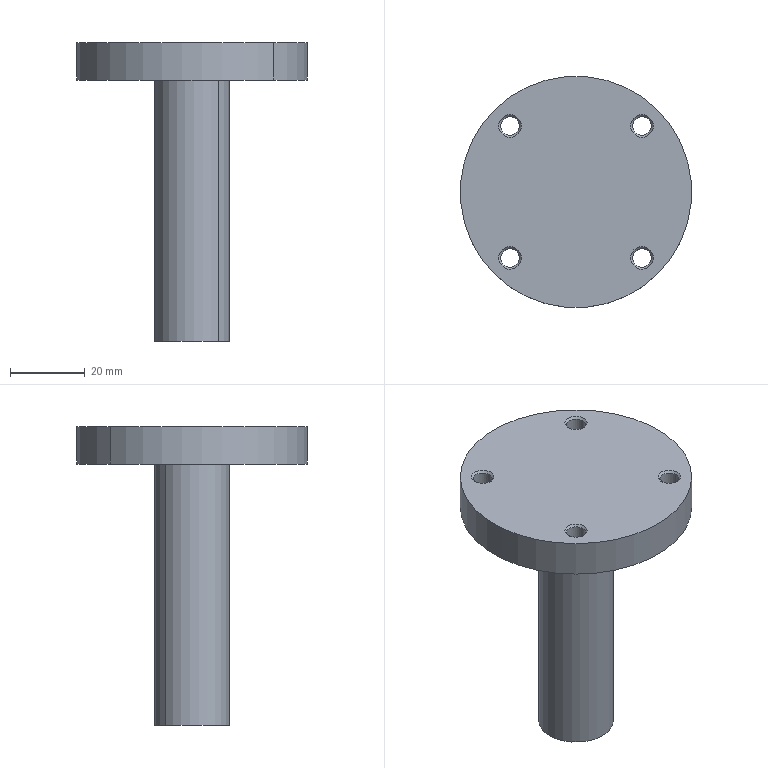Component | SolidWorks | ConnectingBase-3 | 1 solid | 23 faces | box 62 x 62 x 80 mm | volume 51387 mm3 | cylinder 12 | cone 8 | plane 3 | commonest cylinder face diameters 5 x8 20 x2 62 x2
STEP:
#1=COLOUR_RGB('',0.7922,0.8196,0.9333);
#2=FILL_AREA_STYLE_COLOUR('',#1);
#3=FILL_AREA_STYLE('',(#2));
#4=SURFACE_STYLE_FILL_AREA(#3);
#5=SURFACE_SIDE_STYLE('',(#4));
#6=SURFACE_STYLE_USAGE(.BOTH.,#5);
#7=PRESENTATION_STYLE_ASSIGNMENT((#6));
#8=CARTESIAN_POINT('',(-0.4155,17.384,-10.946));
#9=VERTEX_POINT('',#8);
#10=CARTESIAN_POINT('',(-0.5547,17.523,-10.946));
#11=VERTEX_POINT('',#10);
#12=CARTESIAN_POINT('',(-0.4851,17.454,-10.946));
#13=DIRECTION('',(-0.,-0.,1.));
#14=DIRECTION('',(-0.7071,0.7071,0.));
#15=AXIS2_PLACEMENT_3D('',#12,#13,#14);
#16=CIRCLE('',#15,0.09843);
#17=EDGE_CURVE('',#9,#11,#16,.T.);
#18=ORIENTED_EDGE('',*,*,#17,.F.);
#19=CARTESIAN_POINT('',(-0.4009,17.369,-10.925));
#20=VERTEX_POINT('',#19);
#21=CARTESIAN_POINT('',(-0.4155,17.384,-10.946));
#22=DIRECTION('',(0.5,-0.5,0.7071));
#23=VECTOR('',#22,39.37);
#24=LINE('',#21,#23);
#25=EDGE_CURVE('',#9,#20,#24,.T.);
#26=ORIENTED_EDGE('',*,*,#25,.T.);
#27=CARTESIAN_POINT('',(-0.5693,17.538,-10.925));
#28=VERTEX_POINT('',#27);
#29=CARTESIAN_POINT('',(-0.4851,17.454,-10.925));
#30=DIRECTION('',(0.,0.,-1.));
#31=DIRECTION('',(-0.7071,0.7071,0.));
#32=AXIS2_PLACEMENT_3D('',#29,#30,#31);
#33=CIRCLE('',#32,0.1191);
#34=EDGE_CURVE('',#28,#20,#33,.T.);
#35=ORIENTED_EDGE('',*,*,#34,.F.);
#36=CARTESIAN_POINT('',(-0.5547,17.523,-10.946));
#37=DIRECTION('',(-0.5,0.5,0.7071));
#38=VECTOR('',#37,39.37);
#39=LINE('',#36,#38);
#40=EDGE_CURVE('',#11,#28,#39,.T.);
#41=ORIENTED_EDGE('',*,*,#40,.F.);
#42=EDGE_LOOP('',(#18,#26,#35,#41));
#43=FACE_OUTER_BOUND('',#42,.T.);
#44=CARTESIAN_POINT('',(-0.4851,17.454,-10.946));
#45=DIRECTION('',(-0.,-0.,1.));
#46=DIRECTION('',(-0.7071,0.7071,0.));
#47=AXIS2_PLACEMENT_3D('',#44,#45,#46);
#48=CONICAL_SURFACE('',#47,0.09843,0.7854);
#49=ADVANCED_FACE('',(#43),#48,.F.);
#50=CARTESIAN_POINT('',(-1.807,17.384,-10.946));
#51=VERTEX_POINT('',#50);
#52=CARTESIAN_POINT('',(-1.947,17.523,-10.946));
#53=VERTEX_POINT('',#52);
#54=CARTESIAN_POINT('',(-1.877,17.454,-10.946));
#55=DIRECTION('',(-0.,-0.,1.));
#56=DIRECTION('',(-0.7071,0.7071,0.));
#57=AXIS2_PLACEMENT_3D('',#54,#55,#56);
#58=CIRCLE('',#57,0.09843);
#59=EDGE_CURVE('',#51,#53,#58,.T.);
#60=ORIENTED_EDGE('',*,*,#59,.F.);
#61=CARTESIAN_POINT('',(-1.793,17.369,-10.925));
#62=VERTEX_POINT('',#61);
#63=CARTESIAN_POINT('',(-1.807,17.384,-10.946));
#64=DIRECTION('',(0.5,-0.5,0.7071));
#65=VECTOR('',#64,39.37);
#66=LINE('',#63,#65);
#67=EDGE_CURVE('',#51,#62,#66,.T.);
#68=ORIENTED_EDGE('',*,*,#67,.T.);
#69=CARTESIAN_POINT('',(-1.961,17.538,-10.925));
#70=VERTEX_POINT('',#69);
#71=CARTESIAN_POINT('',(-1.877,17.454,-10.925));
#72=DIRECTION('',(0.,0.,-1.));
#73=DIRECTION('',(-0.7071,0.7071,0.));
#74=AXIS2_PLACEMENT_3D('',#71,#72,#73);
#75=CIRCLE('',#74,0.1191);
#76=EDGE_CURVE('',#70,#62,#75,.T.);
#77=ORIENTED_EDGE('',*,*,#76,.F.);
#78=CARTESIAN_POINT('',(-1.947,17.523,-10.946));
#79=DIRECTION('',(-0.5,0.5,0.7071));
#80=VECTOR('',#79,39.37);
#81=LINE('',#78,#80);
#82=EDGE_CURVE('',#53,#70,#81,.T.);
#83=ORIENTED_EDGE('',*,*,#82,.F.);
#84=EDGE_LOOP('',(#60,#68,#77,#83));
#85=FACE_OUTER_BOUND('',#84,.T.);
#86=CARTESIAN_POINT('',(-1.877,17.454,-10.946));
#87=DIRECTION('',(-0.,-0.,1.));
#88=DIRECTION('',(-0.7071,0.7071,0.));
#89=AXIS2_PLACEMENT_3D('',#86,#87,#88);
#90=CONICAL_SURFACE('',#89,0.09843,0.7854);
#91=ADVANCED_FACE('',(#85),#90,.F.);
#92=CARTESIAN_POINT('',(-0.4155,18.776,-10.946));
#93=VERTEX_POINT('',#92);
#94=CARTESIAN_POINT('',(-0.5547,18.915,-10.946));
#95=VERTEX_POINT('',#94);
#96=CARTESIAN_POINT('',(-0.4851,18.846,-10.946));
#97=DIRECTION('',(-0.,-0.,1.));
#98=DIRECTION('',(-0.7071,0.7071,0.));
#99=AXIS2_PLACEMENT_3D('',#96,#97,#98);
#100=CIRCLE('',#99,0.09843);
#101=EDGE_CURVE('',#93,#95,#100,.T.);
#102=ORIENTED_EDGE('',*,*,#101,.F.);
#103=CARTESIAN_POINT('',(-0.4009,18.761,-10.925));
#104=VERTEX_POINT('',#103);
#105=CARTESIAN_POINT('',(-0.4155,18.776,-10.946));
#106=DIRECTION('',(0.5,-0.5,0.7071));
#107=VECTOR('',#106,39.37);
#108=LINE('',#105,#107);
#109=EDGE_CURVE('',#93,#104,#108,.T.);
#110=ORIENTED_EDGE('',*,*,#109,.T.);
#111=CARTESIAN_POINT('',(-0.5693,18.93,-10.925));
#112=VERTEX_POINT('',#111);
#113=CARTESIAN_POINT('',(-0.4851,18.846,-10.925));
#114=DIRECTION('',(0.,0.,-1.));
#115=DIRECTION('',(-0.7071,0.7071,0.));
#116=AXIS2_PLACEMENT_3D('',#113,#114,#115);
#117=CIRCLE('',#116,0.1191);
#118=EDGE_CURVE('',#112,#104,#117,.T.);
#119=ORIENTED_EDGE('',*,*,#118,.F.);
#120=CARTESIAN_POINT('',(-0.5547,18.915,-10.946));
#121=DIRECTION('',(-0.5,0.5,0.7071));
#122=VECTOR('',#121,39.37);
#123=LINE('',#120,#122);
#124=EDGE_CURVE('',#95,#112,#123,.T.);
#125=ORIENTED_EDGE('',*,*,#124,.F.);
#126=EDGE_LOOP('',(#102,#110,#119,#125));
#127=FACE_OUTER_BOUND('',#126,.T.);
#128=CARTESIAN_POINT('',(-0.4851,18.846,-10.946));
#129=DIRECTION('',(-0.,-0.,1.));
#130=DIRECTION('',(-0.7071,0.7071,0.));
#131=AXIS2_PLACEMENT_3D('',#128,#129,#130);
#132=CONICAL_SURFACE('',#131,0.09843,0.7854);
#133=ADVANCED_FACE('',(#127),#132,.F.);
#134=CARTESIAN_POINT('',(-1.807,18.776,-10.946));
#135=VERTEX_POINT('',#134);
#136=CARTESIAN_POINT('',(-1.947,18.915,-10.946));
#137=VERTEX_POINT('',#136);
#138=CARTESIAN_POINT('',(-1.877,18.846,-10.946));
#139=DIRECTION('',(-0.,-0.,1.));
#140=DIRECTION('',(-0.7071,0.7071,0.));
#141=AXIS2_PLACEMENT_3D('',#138,#139,#140);
#142=CIRCLE('',#141,0.09843);
#143=EDGE_CURVE('',#135,#137,#142,.T.);
#144=ORIENTED_EDGE('',*,*,#143,.F.);
#145=CARTESIAN_POINT('',(-1.793,18.761,-10.925));
#146=VERTEX_POINT('',#145);
#147=CARTESIAN_POINT('',(-1.807,18.776,-10.946));
#148=DIRECTION('',(0.5,-0.5,0.7071));
#149=VECTOR('',#148,39.37);
#150=LINE('',#147,#149);
#151=EDGE_CURVE('',#135,#146,#150,.T.);
#152=ORIENTED_EDGE('',*,*,#151,.T.);
#153=CARTESIAN_POINT('',(-1.961,18.93,-10.925));
#154=VERTEX_POINT('',#153);
#155=CARTESIAN_POINT('',(-1.877,18.846,-10.925));
#156=DIRECTION('',(0.,0.,-1.));
#157=DIRECTION('',(-0.7071,0.7071,0.));
#158=AXIS2_PLACEMENT_3D('',#155,#156,#157);
#159=CIRCLE('',#158,0.1191);
#160=EDGE_CURVE('',#154,#146,#159,.T.);
#161=ORIENTED_EDGE('',*,*,#160,.F.);
#162=CARTESIAN_POINT('',(-1.947,18.915,-10.946));
#163=DIRECTION('',(-0.5,0.5,0.7071));
#164=VECTOR('',#163,39.37);
#165=LINE('',#162,#164);
#166=EDGE_CURVE('',#137,#154,#165,.T.);
#167=ORIENTED_EDGE('',*,*,#166,.F.);
#168=EDGE_LOOP('',(#144,#152,#161,#167));
#169=FACE_OUTER_BOUND('',#168,.T.);
#170=CARTESIAN_POINT('',(-1.877,18.846,-10.946));
#171=DIRECTION('',(-0.,-0.,1.));
#172=DIRECTION('',(-0.7071,0.7071,0.));
#173=AXIS2_PLACEMENT_3D('',#170,#171,#172);
#174=CONICAL_SURFACE('',#173,0.09843,0.7854);
#175=ADVANCED_FACE('',(#169),#174,.F.);
#176=CARTESIAN_POINT('',(-1.947,17.523,-11.319));
#177=VERTEX_POINT('',#176);
#178=CARTESIAN_POINT('',(-1.807,17.384,-11.319));
#179=VERTEX_POINT('',#178);
#180=CARTESIAN_POINT('',(-1.877,17.454,-11.319));
#181=DIRECTION('',(0.,0.,-1.));
#182=DIRECTION('',(0.7071,-0.7071,0.));
#183=AXIS2_PLACEMENT_3D('',#180,#181,#182);
#184=CIRCLE('',#183,0.09843);
#185=EDGE_CURVE('',#177,#179,#184,.T.);
#186=ORIENTED_EDGE('',*,*,#185,.T.);
#187=CARTESIAN_POINT('',(-1.807,17.384,-10.925));
#188=DIRECTION('',(-0.,-0.,1.));
#189=VECTOR('',#188,39.37);
#190=LINE('',#187,#189);
#191=EDGE_CURVE('',#179,#51,#190,.T.);
#192=ORIENTED_EDGE('',*,*,#191,.T.);
#193=ORIENTED_EDGE('',*,*,#59,.T.);
#194=CARTESIAN_POINT('',(-1.947,17.523,-10.925));
#195=DIRECTION('',(-0.,-0.,1.));
#196=VECTOR('',#195,39.37);
#197=LINE('',#194,#196);
#198=EDGE_CURVE('',#177,#53,#197,.T.);
#199=ORIENTED_EDGE('',*,*,#198,.F.);
#200=EDGE_LOOP('',(#186,#192,#193,#199));
#201=FACE_OUTER_BOUND('',#200,.T.);
#202=CARTESIAN_POINT('',(-1.877,17.454,-10.925));
#203=DIRECTION('',(-0.,-0.,1.));
#204=DIRECTION('',(-0.7071,0.7071,0.));
#205=AXIS2_PLACEMENT_3D('',#202,#203,#204);
#206=CYLINDRICAL_SURFACE('',#205,0.09843);
#207=ADVANCED_FACE('',(#201),#206,.F.);
#208=CARTESIAN_POINT('',(-0.5547,17.523,-11.319));
#209=VERTEX_POINT('',#208);
#210=CARTESIAN_POINT('',(-0.4155,17.384,-11.319));
#211=VERTEX_POINT('',#210);
#212=CARTESIAN_POINT('',(-0.4851,17.454,-11.319));
#213=DIRECTION('',(0.,0.,-1.));
#214=DIRECTION('',(0.7071,-0.7071,0.));
#215=AXIS2_PLACEMENT_3D('',#212,#213,#214);
#216=CIRCLE('',#215,0.09843);
#217=EDGE_CURVE('',#209,#211,#216,.T.);
#218=ORIENTED_EDGE('',*,*,#217,.T.);
#219=CARTESIAN_POINT('',(-0.4155,17.384,-10.925));
#220=DIRECTION('',(-0.,-0.,1.));
#221=VECTOR('',#220,39.37);
#222=LINE('',#219,#221);
#223=EDGE_CURVE('',#211,#9,#222,.T.);
#224=ORIENTED_EDGE('',*,*,#223,.T.);
#225=ORIENTED_EDGE('',*,*,#17,.T.);
#226=CARTESIAN_POINT('',(-0.5547,17.523,-10.925));
#227=DIRECTION('',(-0.,-0.,1.));
#228=VECTOR('',#227,39.37);
#229=LINE('',#226,#228);
#230=EDGE_CURVE('',#209,#11,#229,.T.);
#231=ORIENTED_EDGE('',*,*,#230,.F.);
#232=EDGE_LOOP('',(#218,#224,#225,#231));
#233=FACE_OUTER_BOUND('',#232,.T.);
#234=CARTESIAN_POINT('',(-0.4851,17.454,-10.925));
#235=DIRECTION('',(-0.,-0.,1.));
#236=DIRECTION('',(-0.7071,0.7071,0.));
#237=AXIS2_PLACEMENT_3D('',#234,#235,#236);
#238=CYLINDRICAL_SURFACE('',#237,0.09843);
#239=ADVANCED_FACE('',(#233),#238,.F.);
#240=CARTESIAN_POINT('',(-0.5547,18.915,-11.319));
#241=VERTEX_POINT('',#240);
#242=CARTESIAN_POINT('',(-0.4155,18.776,-11.319));
#243=VERTEX_POINT('',#242);
#244=CARTESIAN_POINT('',(-0.4851,18.846,-11.319));
#245=DIRECTION('',(0.,0.,-1.));
#246=DIRECTION('',(0.7071,-0.7071,0.));
#247=AXIS2_PLACEMENT_3D('',#244,#245,#246);
#248=CIRCLE('',#247,0.09843);
#249=EDGE_CURVE('',#241,#243,#248,.T.);
#250=ORIENTED_EDGE('',*,*,#249,.T.);
#251=CARTESIAN_POINT('',(-0.4155,18.776,-10.925));
#252=DIRECTION('',(-0.,-0.,1.));
#253=VECTOR('',#252,39.37);
#254=LINE('',#251,#253);
#255=EDGE_CURVE('',#243,#93,#254,.T.);
#256=ORIENTED_EDGE('',*,*,#255,.T.);
#257=ORIENTED_EDGE('',*,*,#101,.T.);
#258=CARTESIAN_POINT('',(-0.5547,18.915,-10.925));
#259=DIRECTION('',(-0.,-0.,1.));
#260=VECTOR('',#259,39.37);
#261=LINE('',#258,#260);
#262=EDGE_CURVE('',#241,#95,#261,.T.);
#263=ORIENTED_EDGE('',*,*,#262,.F.);
#264=EDGE_LOOP('',(#250,#256,#257,#263));
#265=FACE_OUTER_BOUND('',#264,.T.);
#266=CARTESIAN_POINT('',(-0.4851,18.846,-10.925));
#267=DIRECTION('',(-0.,-0.,1.));
#268=DIRECTION('',(-0.7071,0.7071,0.));
#269=AXIS2_PLACEMENT_3D('',#266,#267,#268);
#270=CYLINDRICAL_SURFACE('',#269,0.09843);
#271=ADVANCED_FACE('',(#265),#270,.F.);
#272=CARTESIAN_POINT('',(-1.947,18.915,-11.319));
#273=VERTEX_POINT('',#272);
#274=CARTESIAN_POINT('',(-1.807,18.776,-11.319));
#275=VERTEX_POINT('',#274);
#276=CARTESIAN_POINT('',(-1.877,18.846,-11.319));
#277=DIRECTION('',(0.,0.,-1.));
#278=DIRECTION('',(0.7071,-0.7071,0.));
#279=AXIS2_PLACEMENT_3D('',#276,#277,#278);
#280=CIRCLE('',#279,0.09843);
#281=EDGE_CURVE('',#273,#275,#280,.T.);
#282=ORIENTED_EDGE('',*,*,#281,.T.);
#283=CARTESIAN_POINT('',(-1.807,18.776,-10.925));
#284=DIRECTION('',(-0.,-0.,1.));
#285=VECTOR('',#284,39.37);
#286=LINE('',#283,#285);
#287=EDGE_CURVE('',#275,#135,#286,.T.);
#288=ORIENTED_EDGE('',*,*,#287,.T.);
#289=ORIENTED_EDGE('',*,*,#143,.T.);
#290=CARTESIAN_POINT('',(-1.947,18.915,-10.925));
#291=DIRECTION('',(-0.,-0.,1.));
#292=VECTOR('',#291,39.37);
#293=LINE('',#290,#292);
#294=EDGE_CURVE('',#273,#137,#293,.T.);
#295=ORIENTED_EDGE('',*,*,#294,.F.);
#296=EDGE_LOOP('',(#282,#288,#289,#295));
#297=FACE_OUTER_BOUND('',#296,.T.);
#298=CARTESIAN_POINT('',(-1.877,18.846,-10.925));
#299=DIRECTION('',(-0.,-0.,1.));
#300=DIRECTION('',(-0.7071,0.7071,0.));
#301=AXIS2_PLACEMENT_3D('',#298,#299,#300);
#302=CYLINDRICAL_SURFACE('',#301,0.09843);
#303=ADVANCED_FACE('',(#297),#302,.F.);
#304=CARTESIAN_POINT('',(-0.9027,17.871,-14.075));
#305=VERTEX_POINT('',#304);
#306=CARTESIAN_POINT('',(-1.459,18.428,-14.075));
#307=VERTEX_POINT('',#306);
#308=CARTESIAN_POINT('',(-1.181,18.15,-14.075));
#309=DIRECTION('',(0.,0.,-1.));
#310=DIRECTION('',(0.7071,-0.7071,0.));
#311=AXIS2_PLACEMENT_3D('',#308,#309,#310);
#312=CIRCLE('',#311,0.3937);
#313=EDGE_CURVE('',#305,#307,#312,.T.);
#314=ORIENTED_EDGE('',*,*,#313,.F.);
#315=CARTESIAN_POINT('',(-0.9027,17.871,-11.319));
#316=VERTEX_POINT('',#315);
#317=CARTESIAN_POINT('',(-0.9027,17.871,-14.075));
#318=DIRECTION('',(-0.,-0.,1.));
#319=VECTOR('',#318,39.37);
#320=LINE('',#317,#319);
#321=EDGE_CURVE('',#305,#316,#320,.T.);
#322=ORIENTED_EDGE('',*,*,#321,.T.);
#323=CARTESIAN_POINT('',(-1.459,18.428,-11.319));
#324=VERTEX_POINT('',#323);
#325=CARTESIAN_POINT('',(-1.181,18.15,-11.319));
#326=DIRECTION('',(0.,0.,-1.));
#327=DIRECTION('',(0.7071,-0.7071,0.));
#328=AXIS2_PLACEMENT_3D('',#325,#326,#327);
#329=CIRCLE('',#328,0.3937);
#330=EDGE_CURVE('',#316,#324,#329,.T.);
#331=ORIENTED_EDGE('',*,*,#330,.T.);
#332=CARTESIAN_POINT('',(-1.459,18.428,-14.075));
#333=DIRECTION('',(-0.,-0.,1.));
#334=VECTOR('',#333,39.37);
#335=LINE('',#332,#334);
#336=EDGE_CURVE('',#307,#324,#335,.T.);
#337=ORIENTED_EDGE('',*,*,#336,.F.);
#338=EDGE_LOOP('',(#314,#322,#331,#337));
#339=FACE_OUTER_BOUND('',#338,.T.);
#340=CARTESIAN_POINT('',(-1.181,18.15,-14.075));
#341=DIRECTION('',(-0.,-0.,1.));
#342=DIRECTION('',(-0.7071,0.7071,0.));
#343=AXIS2_PLACEMENT_3D('',#340,#341,#342);
#344=CYLINDRICAL_SURFACE('',#343,0.3937);
#345=ADVANCED_FACE('',(#339),#344,.T.);
#346=CARTESIAN_POINT('',(-2.044,19.013,-11.319));
#347=VERTEX_POINT('',#346);
#348=CARTESIAN_POINT('',(-0.3181,17.287,-11.319));
#349=VERTEX_POINT('',#348);
#350=CARTESIAN_POINT('',(-1.181,18.15,-11.319));
#351=DIRECTION('',(-0.,-0.,1.));
#352=DIRECTION('',(-0.7071,0.7071,0.));
#353=AXIS2_PLACEMENT_3D('',#350,#351,#352);
#354=CIRCLE('',#353,1.22);
#355=EDGE_CURVE('',#347,#349,#354,.T.);
#356=ORIENTED_EDGE('',*,*,#355,.T.);
#357=CARTESIAN_POINT('',(-0.3181,17.287,-10.925));
#358=VERTEX_POINT('',#357);
#359=CARTESIAN_POINT('',(-0.3181,17.287,-11.319));
#360=DIRECTION('',(-0.,-0.,1.));
#361=VECTOR('',#360,39.37);
#362=LINE('',#359,#361);
#363=EDGE_CURVE('',#349,#358,#362,.T.);
#364=ORIENTED_EDGE('',*,*,#363,.T.);
#365=CARTESIAN_POINT('',(-2.044,19.013,-10.925));
#366=VERTEX_POINT('',#365);
#367=CARTESIAN_POINT('',(-1.181,18.15,-10.925));
#368=DIRECTION('',(-0.,-0.,1.));
#369=DIRECTION('',(-0.7071,0.7071,0.));
#370=AXIS2_PLACEMENT_3D('',#367,#368,#369);
#371=CIRCLE('',#370,1.22);
#372=EDGE_CURVE('',#366,#358,#371,.T.);
#373=ORIENTED_EDGE('',*,*,#372,.F.);
#374=CARTESIAN_POINT('',(-2.044,19.013,-11.319));
#375=DIRECTION('',(-0.,-0.,1.));
#376=VECTOR('',#375,39.37);
#377=LINE('',#374,#376);
#378=EDGE_CURVE('',#347,#366,#377,.T.);
#379=ORIENTED_EDGE('',*,*,#378,.F.);
#380=EDGE_LOOP('',(#356,#364,#373,#379));
#381=FACE_OUTER_BOUND('',#380,.T.);
#382=CARTESIAN_POINT('',(-1.181,18.15,-11.319));
#383=DIRECTION('',(-0.,-0.,1.));
#384=DIRECTION('',(-0.7071,0.7071,0.));
#385=AXIS2_PLACEMENT_3D('',#382,#383,#384);
#386=CYLINDRICAL_SURFACE('',#385,1.22);
#387=ADVANCED_FACE('',(#381),#386,.T.);
#388=ORIENTED_EDGE('',*,*,#363,.F.);
#389=CARTESIAN_POINT('',(-1.181,18.15,-11.319));
#390=DIRECTION('',(-0.,-0.,1.));
#391=DIRECTION('',(-0.7071,0.7071,0.));
#392=AXIS2_PLACEMENT_3D('',#389,#390,#391);
#393=CIRCLE('',#392,1.22);
#394=EDGE_CURVE('',#349,#347,#393,.T.);
#395=ORIENTED_EDGE('',*,*,#394,.T.);
#396=ORIENTED_EDGE('',*,*,#378,.T.);
#397=CARTESIAN_POINT('',(-1.181,18.15,-10.925));
#398=DIRECTION('',(-0.,-0.,1.));
#399=DIRECTION('',(-0.7071,0.7071,0.));
#400=AXIS2_PLACEMENT_3D('',#397,#398,#399);
#401=CIRCLE('',#400,1.22);
#402=EDGE_CURVE('',#358,#366,#401,.T.);
#403=ORIENTED_EDGE('',*,*,#402,.F.);
#404=EDGE_LOOP('',(#388,#395,#396,#403));
#405=FACE_OUTER_BOUND('',#404,.T.);
#406=CARTESIAN_POINT('',(-1.181,18.15,-11.319));
#407=DIRECTION('',(-0.,-0.,1.));
#408=DIRECTION('',(-0.7071,0.7071,0.));
#409=AXIS2_PLACEMENT_3D('',#406,#407,#408);
#410=CYLINDRICAL_SURFACE('',#409,1.22);
#411=ADVANCED_FACE('',(#405),#410,.T.);
#412=ORIENTED_EDGE('',*,*,#185,.F.);
#413=CARTESIAN_POINT('',(-1.877,17.454,-11.319));
#414=DIRECTION('',(0.,0.,-1.));
#415=DIRECTION('',(0.7071,-0.7071,0.));
#416=AXIS2_PLACEMENT_3D('',#413,#414,#415);
#417=CIRCLE('',#416,0.09843);
#418=EDGE_CURVE('',#179,#177,#417,.T.);
#419=ORIENTED_EDGE('',*,*,#418,.F.);
#420=EDGE_LOOP('',(#412,#419));
#421=FACE_BOUND('',#420,.T.);
#422=ORIENTED_EDGE('',*,*,#217,.F.);
#423=CARTESIAN_POINT('',(-0.4851,17.454,-11.319));
#424=DIRECTION('',(0.,0.,-1.));
#425=DIRECTION('',(0.7071,-0.7071,0.));
#426=AXIS2_PLACEMENT_3D('',#423,#424,#425);
#427=CIRCLE('',#426,0.09843);
#428=EDGE_CURVE('',#211,#209,#427,.T.);
#429=ORIENTED_EDGE('',*,*,#428,.F.);
#430=EDGE_LOOP('',(#422,#429));
#431=FACE_BOUND('',#430,.T.);
#432=ORIENTED_EDGE('',*,*,#249,.F.);
#433=CARTESIAN_POINT('',(-0.4851,18.846,-11.319));
#434=DIRECTION('',(0.,0.,-1.));
#435=DIRECTION('',(0.7071,-0.7071,0.));
#436=AXIS2_PLACEMENT_3D('',#433,#434,#435);
#437=CIRCLE('',#436,0.09843);
#438=EDGE_CURVE('',#243,#241,#437,.T.);
#439=ORIENTED_EDGE('',*,*,#438,.F.);
#440=EDGE_LOOP('',(#432,#439));
#441=FACE_BOUND('',#440,.T.);
#442=ORIENTED_EDGE('',*,*,#281,.F.);
#443=CARTESIAN_POINT('',(-1.877,18.846,-11.319));
#444=DIRECTION('',(0.,0.,-1.));
#445=DIRECTION('',(0.7071,-0.7071,0.));
#446=AXIS2_PLACEMENT_3D('',#443,#444,#445);
#447=CIRCLE('',#446,0.09843);
#448=EDGE_CURVE('',#275,#273,#447,.T.);
#449=ORIENTED_EDGE('',*,*,#448,.F.);
#450=EDGE_LOOP('',(#442,#449));
#451=FACE_BOUND('',#450,.T.);
#452=CARTESIAN_POINT('',(-1.181,18.15,-11.319));
#453=DIRECTION('',(0.,0.,-1.));
#454=DIRECTION('',(0.7071,-0.7071,0.));
#455=AXIS2_PLACEMENT_3D('',#452,#453,#454);
#456=CIRCLE('',#455,0.3937);
#457=EDGE_CURVE('',#324,#316,#456,.T.);
#458=ORIENTED_EDGE('',*,*,#457,.F.);
#459=ORIENTED_EDGE('',*,*,#330,.F.);
#460=EDGE_LOOP('',(#458,#459));
#461=FACE_BOUND('',#460,.T.);
#462=ORIENTED_EDGE('',*,*,#355,.F.);
#463=ORIENTED_EDGE('',*,*,#394,.F.);
#464=EDGE_LOOP('',(#462,#463));
#465=FACE_OUTER_BOUND('',#464,.T.);
#466=CARTESIAN_POINT('',(-2.044,17.287,-11.319));
#467=DIRECTION('',(0.,0.,-1.));
#468=DIRECTION('',(0.7071,-0.7071,0.));
#469=AXIS2_PLACEMENT_3D('',#466,#467,#468);
#470=PLANE('',#469);
#471=ADVANCED_FACE('',(#421,#431,#441,#451,#461,#465),#470,.T.);
#472=ORIENTED_EDGE('',*,*,#160,.T.);
#473=CARTESIAN_POINT('',(-1.877,18.846,-10.925));
#474=DIRECTION('',(0.,0.,-1.));
#475=DIRECTION('',(-0.7071,0.7071,0.));
#476=AXIS2_PLACEMENT_3D('',#473,#474,#475);
#477=CIRCLE('',#476,0.1191);
#478=EDGE_CURVE('',#146,#154,#477,.T.);
#479=ORIENTED_EDGE('',*,*,#478,.T.);
#480=EDGE_LOOP('',(#472,#479));
#481=FACE_BOUND('',#480,.T.);
#482=ORIENTED_EDGE('',*,*,#118,.T.);
#483=CARTESIAN_POINT('',(-0.4851,18.846,-10.925));
#484=DIRECTION('',(0.,0.,-1.));
#485=DIRECTION('',(-0.7071,0.7071,0.));
#486=AXIS2_PLACEMENT_3D('',#483,#484,#485);
#487=CIRCLE('',#486,0.1191);
#488=EDGE_CURVE('',#104,#112,#487,.T.);
#489=ORIENTED_EDGE('',*,*,#488,.T.);
#490=EDGE_LOOP('',(#482,#489));
#491=FACE_BOUND('',#490,.T.);
#492=ORIENTED_EDGE('',*,*,#76,.T.);
#493=CARTESIAN_POINT('',(-1.877,17.454,-10.925));
#494=DIRECTION('',(0.,0.,-1.));
#495=DIRECTION('',(-0.7071,0.7071,0.));
#496=AXIS2_PLACEMENT_3D('',#493,#494,#495);
#497=CIRCLE('',#496,0.1191);
#498=EDGE_CURVE('',#62,#70,#497,.T.);
#499=ORIENTED_EDGE('',*,*,#498,.T.);
#500=EDGE_LOOP('',(#492,#499));
#501=FACE_BOUND('',#500,.T.);
#502=ORIENTED_EDGE('',*,*,#34,.T.);
#503=CARTESIAN_POINT('',(-0.4851,17.454,-10.925));
#504=DIRECTION('',(0.,0.,-1.));
#505=DIRECTION('',(-0.7071,0.7071,0.));
#506=AXIS2_PLACEMENT_3D('',#503,#504,#505);
#507=CIRCLE('',#506,0.1191);
#508=EDGE_CURVE('',#20,#28,#507,.T.);
#509=ORIENTED_EDGE('',*,*,#508,.T.);
#510=EDGE_LOOP('',(#502,#509));
#511=FACE_BOUND('',#510,.T.);
#512=ORIENTED_EDGE('',*,*,#372,.T.);
#513=ORIENTED_EDGE('',*,*,#402,.T.);
#514=EDGE_LOOP('',(#512,#513));
#515=FACE_OUTER_BOUND('',#514,.T.);
#516=CARTESIAN_POINT('',(-1.181,18.15,-10.925));
#517=DIRECTION('',(-0.,-0.,1.));
#518=DIRECTION('',(-0.7071,0.7071,0.));
#519=AXIS2_PLACEMENT_3D('',#516,#517,#518);
#520=PLANE('',#519);
#521=ADVANCED_FACE('',(#481,#491,#501,#511,#515),#520,.T.);
#522=ORIENTED_EDGE('',*,*,#321,.F.);
#523=CARTESIAN_POINT('',(-1.181,18.15,-14.075));
#524=DIRECTION('',(0.,0.,-1.));
#525=DIRECTION('',(0.7071,-0.7071,0.));
#526=AXIS2_PLACEMENT_3D('',#523,#524,#525);
#527=CIRCLE('',#526,0.3937);
#528=EDGE_CURVE('',#307,#305,#527,.T.);
#529=ORIENTED_EDGE('',*,*,#528,.F.);
#530=ORIENTED_EDGE('',*,*,#336,.T.);
#531=ORIENTED_EDGE('',*,*,#457,.T.);
#532=EDGE_LOOP('',(#522,#529,#530,#531));
#533=FACE_OUTER_BOUND('',#532,.T.);
#534=CARTESIAN_POINT('',(-1.181,18.15,-14.075));
#535=DIRECTION('',(-0.,-0.,1.));
#536=DIRECTION('',(-0.7071,0.7071,0.));
#537=AXIS2_PLACEMENT_3D('',#534,#535,#536);
#538=CYLINDRICAL_SURFACE('',#537,0.3937);
#539=ADVANCED_FACE('',(#533),#538,.T.);
#540=ORIENTED_EDGE('',*,*,#528,.T.);
#541=ORIENTED_EDGE('',*,*,#313,.T.);
#542=EDGE_LOOP('',(#540,#541));
#543=FACE_OUTER_BOUND('',#542,.T.);
#544=CARTESIAN_POINT('',(-1.181,18.15,-14.075));
#545=DIRECTION('',(0.,0.,-1.));
#546=DIRECTION('',(0.7071,-0.7071,0.));
#547=AXIS2_PLACEMENT_3D('',#544,#545,#546);
#548=PLANE('',#547);
#549=ADVANCED_FACE('',(#543),#548,.T.);
#550=ORIENTED_EDGE('',*,*,#287,.F.);
#551=ORIENTED_EDGE('',*,*,#448,.T.);
#552=ORIENTED_EDGE('',*,*,#294,.T.);
#553=CARTESIAN_POINT('',(-1.877,18.846,-10.946));
#554=DIRECTION('',(-0.,-0.,1.));
#555=DIRECTION('',(-0.7071,0.7071,0.));
#556=AXIS2_PLACEMENT_3D('',#553,#554,#555);
#557=CIRCLE('',#556,0.09843);
#558=EDGE_CURVE('',#137,#135,#557,.T.);
#559=ORIENTED_EDGE('',*,*,#558,.T.);
#560=EDGE_LOOP('',(#550,#551,#552,#559));
#561=FACE_OUTER_BOUND('',#560,.T.);
#562=CARTESIAN_POINT('',(-1.877,18.846,-10.925));
#563=DIRECTION('',(-0.,-0.,1.));
#564=DIRECTION('',(-0.7071,0.7071,0.));
#565=AXIS2_PLACEMENT_3D('',#562,#563,#564);
#566=CYLINDRICAL_SURFACE('',#565,0.09843);
#567=ADVANCED_FACE('',(#561),#566,.F.);
#568=ORIENTED_EDGE('',*,*,#255,.F.);
#569=ORIENTED_EDGE('',*,*,#438,.T.);
#570=ORIENTED_EDGE('',*,*,#262,.T.);
#571=CARTESIAN_POINT('',(-0.4851,18.846,-10.946));
#572=DIRECTION('',(-0.,-0.,1.));
#573=DIRECTION('',(-0.7071,0.7071,0.));
#574=AXIS2_PLACEMENT_3D('',#571,#572,#573);
#575=CIRCLE('',#574,0.09843);
#576=EDGE_CURVE('',#95,#93,#575,.T.);
#577=ORIENTED_EDGE('',*,*,#576,.T.);
#578=EDGE_LOOP('',(#568,#569,#570,#577));
#579=FACE_OUTER_BOUND('',#578,.T.);
#580=CARTESIAN_POINT('',(-0.4851,18.846,-10.925));
#581=DIRECTION('',(-0.,-0.,1.));
#582=DIRECTION('',(-0.7071,0.7071,0.));
#583=AXIS2_PLACEMENT_3D('',#580,#581,#582);
#584=CYLINDRICAL_SURFACE('',#583,0.09843);
#585=ADVANCED_FACE('',(#579),#584,.F.);
#586=ORIENTED_EDGE('',*,*,#223,.F.);
#587=ORIENTED_EDGE('',*,*,#428,.T.);
#588=ORIENTED_EDGE('',*,*,#230,.T.);
#589=CARTESIAN_POINT('',(-0.4851,17.454,-10.946));
#590=DIRECTION('',(-0.,-0.,1.));
#591=DIRECTION('',(-0.7071,0.7071,0.));
#592=AXIS2_PLACEMENT_3D('',#589,#590,#591);
#593=CIRCLE('',#592,0.09843);
#594=EDGE_CURVE('',#11,#9,#593,.T.);
#595=ORIENTED_EDGE('',*,*,#594,.T.);
#596=EDGE_LOOP('',(#586,#587,#588,#595));
#597=FACE_OUTER_BOUND('',#596,.T.);
#598=CARTESIAN_POINT('',(-0.4851,17.454,-10.925));
#599=DIRECTION('',(-0.,-0.,1.));
#600=DIRECTION('',(-0.7071,0.7071,0.));
#601=AXIS2_PLACEMENT_3D('',#598,#599,#600);
#602=CYLINDRICAL_SURFACE('',#601,0.09843);
#603=ADVANCED_FACE('',(#597),#602,.F.);
#604=ORIENTED_EDGE('',*,*,#191,.F.);
#605=ORIENTED_EDGE('',*,*,#418,.T.);
#606=ORIENTED_EDGE('',*,*,#198,.T.);
#607=CARTESIAN_POINT('',(-1.877,17.454,-10.946));
#608=DIRECTION('',(-0.,-0.,1.));
#609=DIRECTION('',(-0.7071,0.7071,0.));
#610=AXIS2_PLACEMENT_3D('',#607,#608,#609);
#611=CIRCLE('',#610,0.09843);
#612=EDGE_CURVE('',#53,#51,#611,.T.);
#613=ORIENTED_EDGE('',*,*,#612,.T.);
#614=EDGE_LOOP('',(#604,#605,#606,#613));
#615=FACE_OUTER_BOUND('',#614,.T.);
#616=CARTESIAN_POINT('',(-1.877,17.454,-10.925));
#617=DIRECTION('',(-0.,-0.,1.));
#618=DIRECTION('',(-0.7071,0.7071,0.));
#619=AXIS2_PLACEMENT_3D('',#616,#617,#618);
#620=CYLINDRICAL_SURFACE('',#619,0.09843);
#621=ADVANCED_FACE('',(#615),#620,.F.);
#622=ORIENTED_EDGE('',*,*,#151,.F.);
#623=ORIENTED_EDGE('',*,*,#558,.F.);
#624=ORIENTED_EDGE('',*,*,#166,.T.);
#625=ORIENTED_EDGE('',*,*,#478,.F.);
#626=EDGE_LOOP('',(#622,#623,#624,#625));
#627=FACE_OUTER_BOUND('',#626,.T.);
#628=CARTESIAN_POINT('',(-1.877,18.846,-10.946));
#629=DIRECTION('',(-0.,-0.,1.));
#630=DIRECTION('',(-0.7071,0.7071,0.));
#631=AXIS2_PLACEMENT_3D('',#628,#629,#630);
#632=CONICAL_SURFACE('',#631,0.09843,0.7854);
#633=ADVANCED_FACE('',(#627),#632,.F.);
#634=ORIENTED_EDGE('',*,*,#109,.F.);
#635=ORIENTED_EDGE('',*,*,#576,.F.);
#636=ORIENTED_EDGE('',*,*,#124,.T.);
#637=ORIENTED_EDGE('',*,*,#488,.F.);
#638=EDGE_LOOP('',(#634,#635,#636,#637));
#639=FACE_OUTER_BOUND('',#638,.T.);
#640=CARTESIAN_POINT('',(-0.4851,18.846,-10.946));
#641=DIRECTION('',(-0.,-0.,1.));
#642=DIRECTION('',(-0.7071,0.7071,0.));
#643=AXIS2_PLACEMENT_3D('',#640,#641,#642);
#644=CONICAL_SURFACE('',#643,0.09843,0.7854);
#645=ADVANCED_FACE('',(#639),#644,.F.);
#646=ORIENTED_EDGE('',*,*,#67,.F.);
#647=ORIENTED_EDGE('',*,*,#612,.F.);
#648=ORIENTED_EDGE('',*,*,#82,.T.);
#649=ORIENTED_EDGE('',*,*,#498,.F.);
#650=EDGE_LOOP('',(#646,#647,#648,#649));
#651=FACE_OUTER_BOUND('',#650,.T.);
#652=CARTESIAN_POINT('',(-1.877,17.454,-10.946));
#653=DIRECTION('',(-0.,-0.,1.));
#654=DIRECTION('',(-0.7071,0.7071,0.));
#655=AXIS2_PLACEMENT_3D('',#652,#653,#654);
#656=CONICAL_SURFACE('',#655,0.09843,0.7854);
#657=ADVANCED_FACE('',(#651),#656,.F.);
#658=ORIENTED_EDGE('',*,*,#25,.F.);
#659=ORIENTED_EDGE('',*,*,#594,.F.);
#660=ORIENTED_EDGE('',*,*,#40,.T.);
#661=ORIENTED_EDGE('',*,*,#508,.F.);
#662=EDGE_LOOP('',(#658,#659,#660,#661));
#663=FACE_OUTER_BOUND('',#662,.T.);
#664=CARTESIAN_POINT('',(-0.4851,17.454,-10.946));
#665=DIRECTION('',(-0.,-0.,1.));
#666=DIRECTION('',(-0.7071,0.7071,0.));
#667=AXIS2_PLACEMENT_3D('',#664,#665,#666);
#668=CONICAL_SURFACE('',#667,0.09843,0.7854);
#669=ADVANCED_FACE('',(#663),#668,.F.);
#670=CLOSED_SHELL('',(#49,#91,#133,#175,#207,#239,#271,#303,#345,#387,#411,#471,#521,#539,#549,#567,#585,#603,#621,#633,#645,#657,#669));
#671=MANIFOLD_SOLID_BREP('',#670);
#672=STYLED_ITEM('',(#7),#671);
#673=PRESENTATION_LAYER_ASSIGNMENT('','',(#672));
#674=CARTESIAN_POINT('',(0.,0.,0.));
#675=DIRECTION('',(0.,0.,1.));
#676=DIRECTION('',(1.,0.,0.));
#677=AXIS2_PLACEMENT_3D('',#674,#675,#676);
#678=(LENGTH_UNIT()NAMED_UNIT(*)SI_UNIT($,.METRE.));
#679=LENGTH_MEASURE_WITH_UNIT(LENGTH_MEASURE(0.0254),#678);
#680=DIMENSIONAL_EXPONENTS(1.,0.,0.,0.,0.,0.,0.);
#681=(CONVERSION_BASED_UNIT('',#679)LENGTH_UNIT()NAMED_UNIT(#680));
#682=UNCERTAINTY_MEASURE_WITH_UNIT(LENGTH_MEASURE(0.00001),#681,'','');
#683=(NAMED_UNIT(*)PLANE_ANGLE_UNIT()SI_UNIT($,.RADIAN.));
#684=(NAMED_UNIT(*)SI_UNIT($,.STERADIAN.)SOLID_ANGLE_UNIT());
#685=(GEOMETRIC_REPRESENTATION_CONTEXT(3)GLOBAL_UNCERTAINTY_ASSIGNED_CONTEXT((#682))GLOBAL_UNIT_ASSIGNED_CONTEXT((#681,#683,#684))REPRESENTATION_CONTEXT('',''));
#686=ADVANCED_BREP_SHAPE_REPRESENTATION('',(#671,#677),#685);
#687=(LENGTH_UNIT()NAMED_UNIT(*)SI_UNIT($,.METRE.));
#688=LENGTH_MEASURE_WITH_UNIT(LENGTH_MEASURE(0.0254),#687);
#689=DIMENSIONAL_EXPONENTS(1.,0.,0.,0.,0.,0.,0.);
#690=(CONVERSION_BASED_UNIT('',#688)LENGTH_UNIT()NAMED_UNIT(#689));
#691=UNCERTAINTY_MEASURE_WITH_UNIT(LENGTH_MEASURE(0.00001),#690,'','');
#692=(NAMED_UNIT(*)PLANE_ANGLE_UNIT()SI_UNIT($,.RADIAN.));
#693=(NAMED_UNIT(*)SI_UNIT($,.STERADIAN.)SOLID_ANGLE_UNIT());
#694=(GEOMETRIC_REPRESENTATION_CONTEXT(3)GLOBAL_UNCERTAINTY_ASSIGNED_CONTEXT((#691))GLOBAL_UNIT_ASSIGNED_CONTEXT((#690,#692,#693))REPRESENTATION_CONTEXT('',''));
#695=MECHANICAL_DESIGN_GEOMETRIC_PRESENTATION_REPRESENTATION('',(#672),#694);